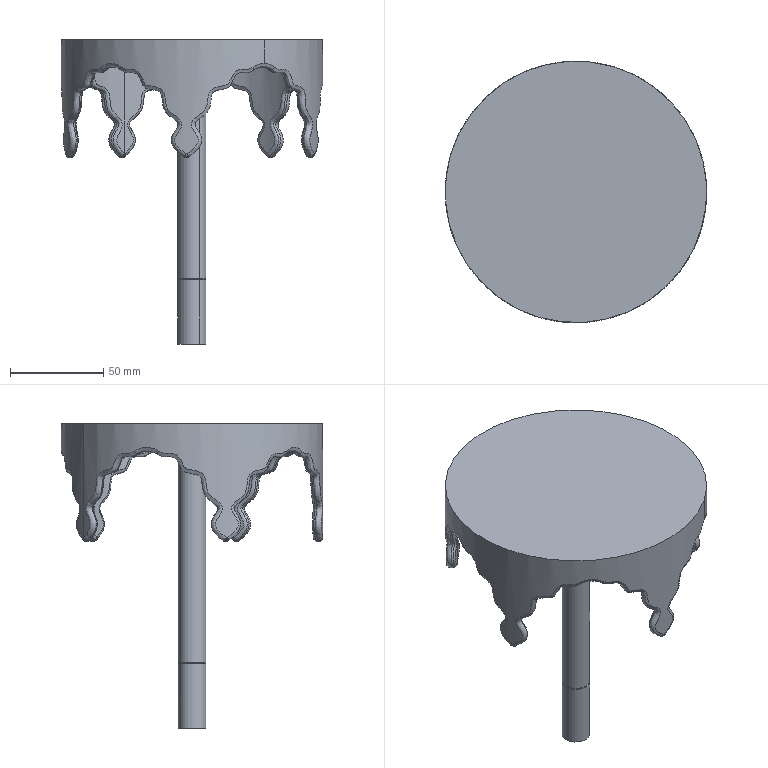Component | SolidWorks | FormingWheel-2 | 1 solid | 123 faces | volume 130022 mm3 | spline 45 | sphere 32 | cylinder 26 | plane 14 | torus 6 | commonest cylinder face diameters 4 x10 20 x6 15 x4 14.5 x2 130 x2 140 x2